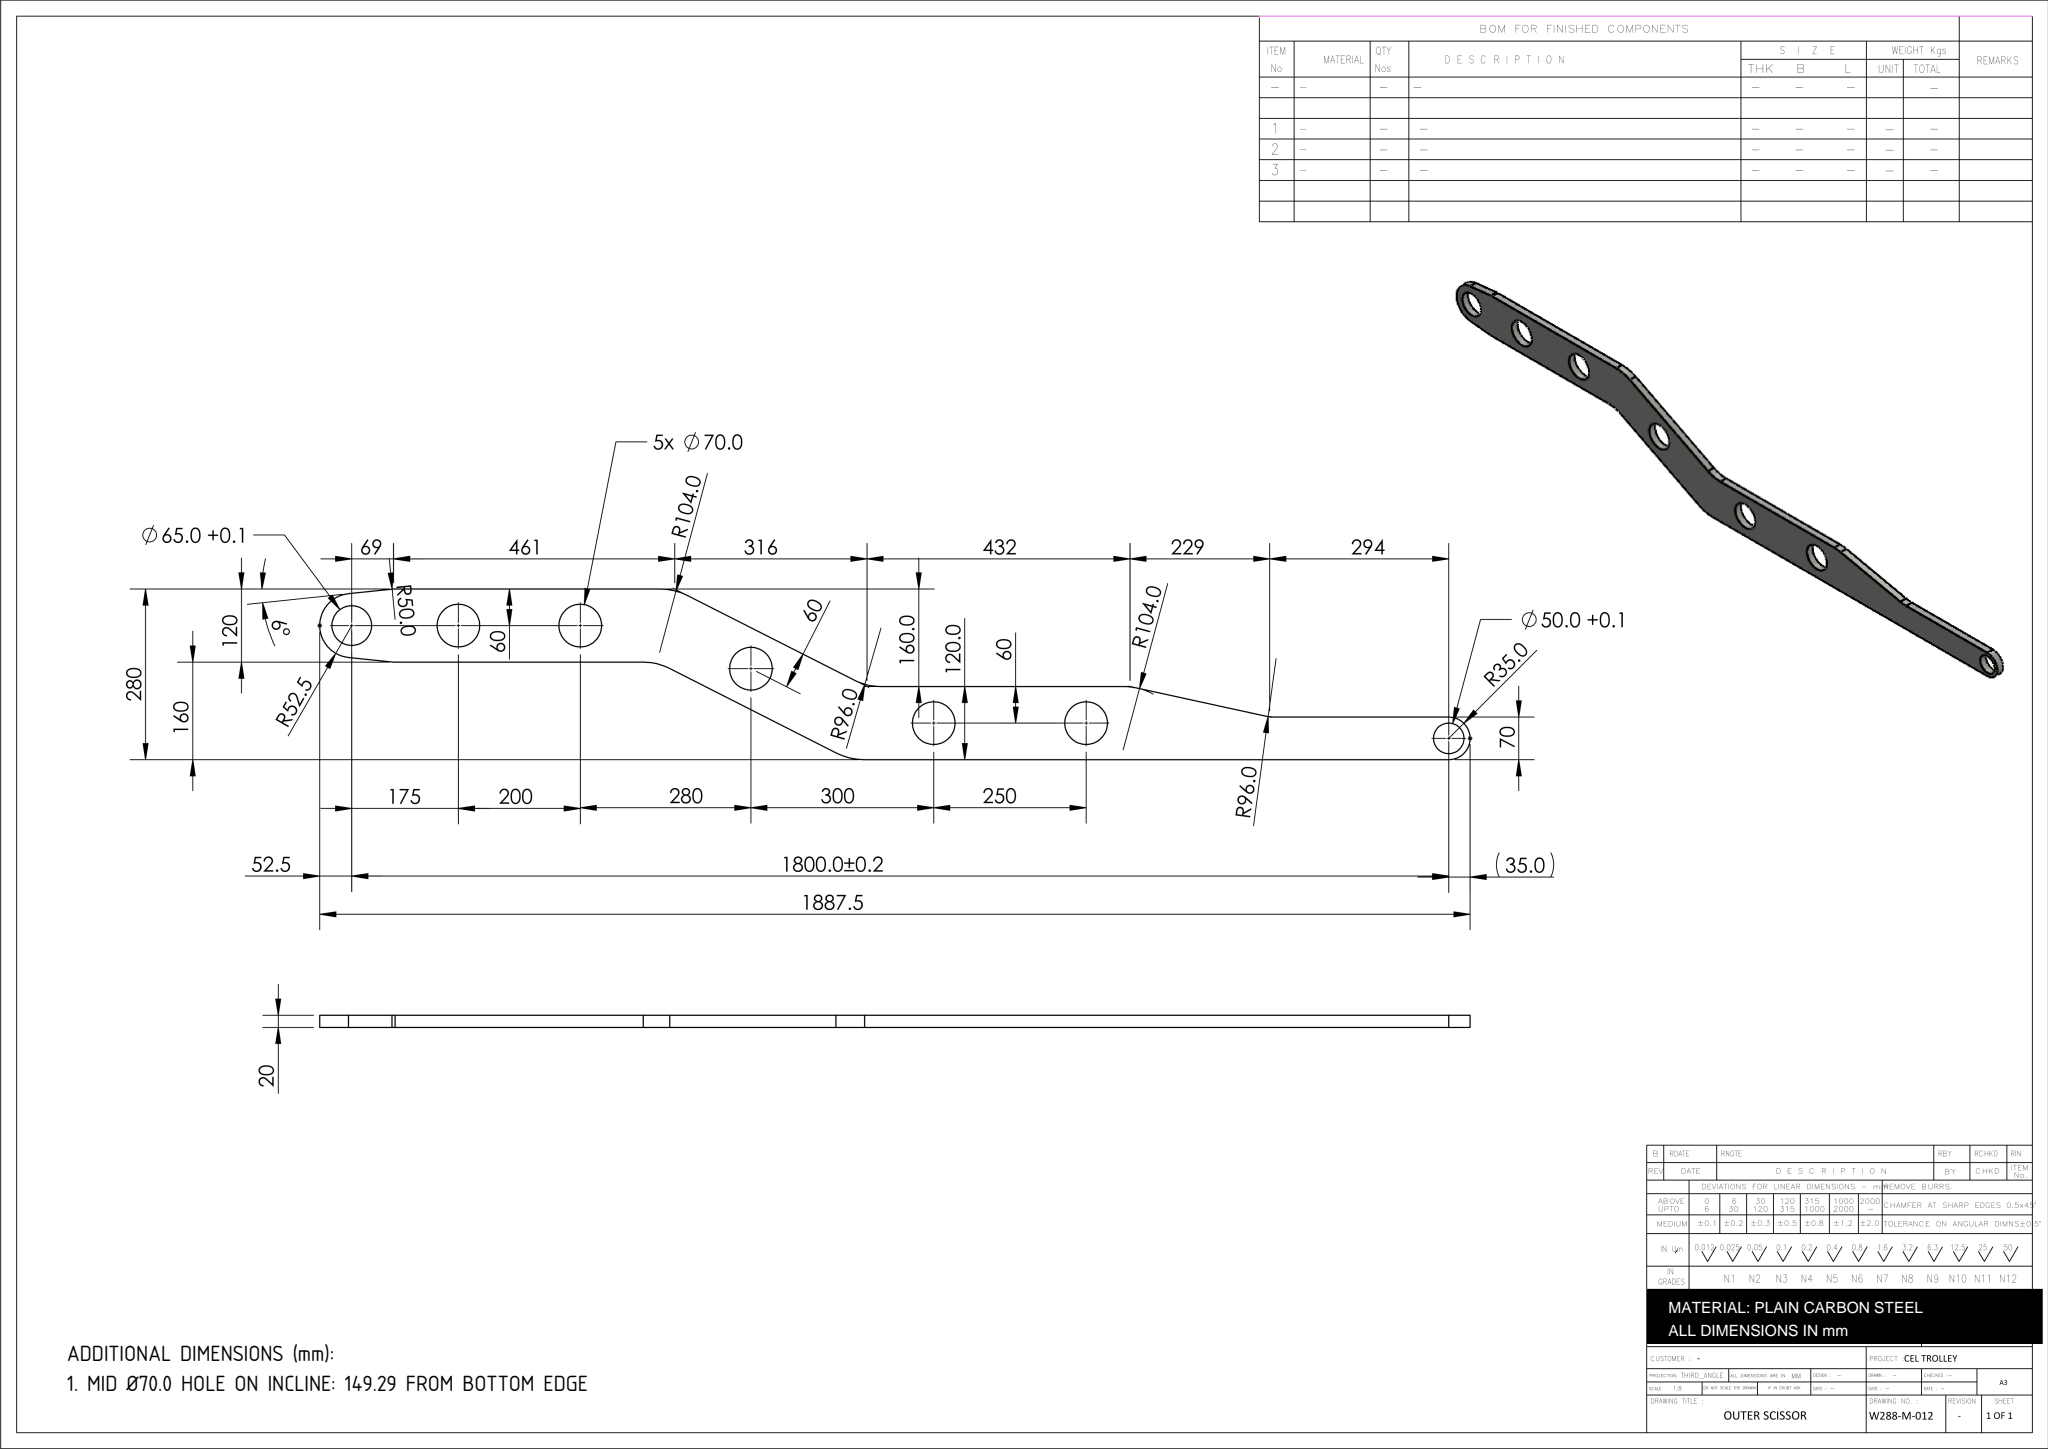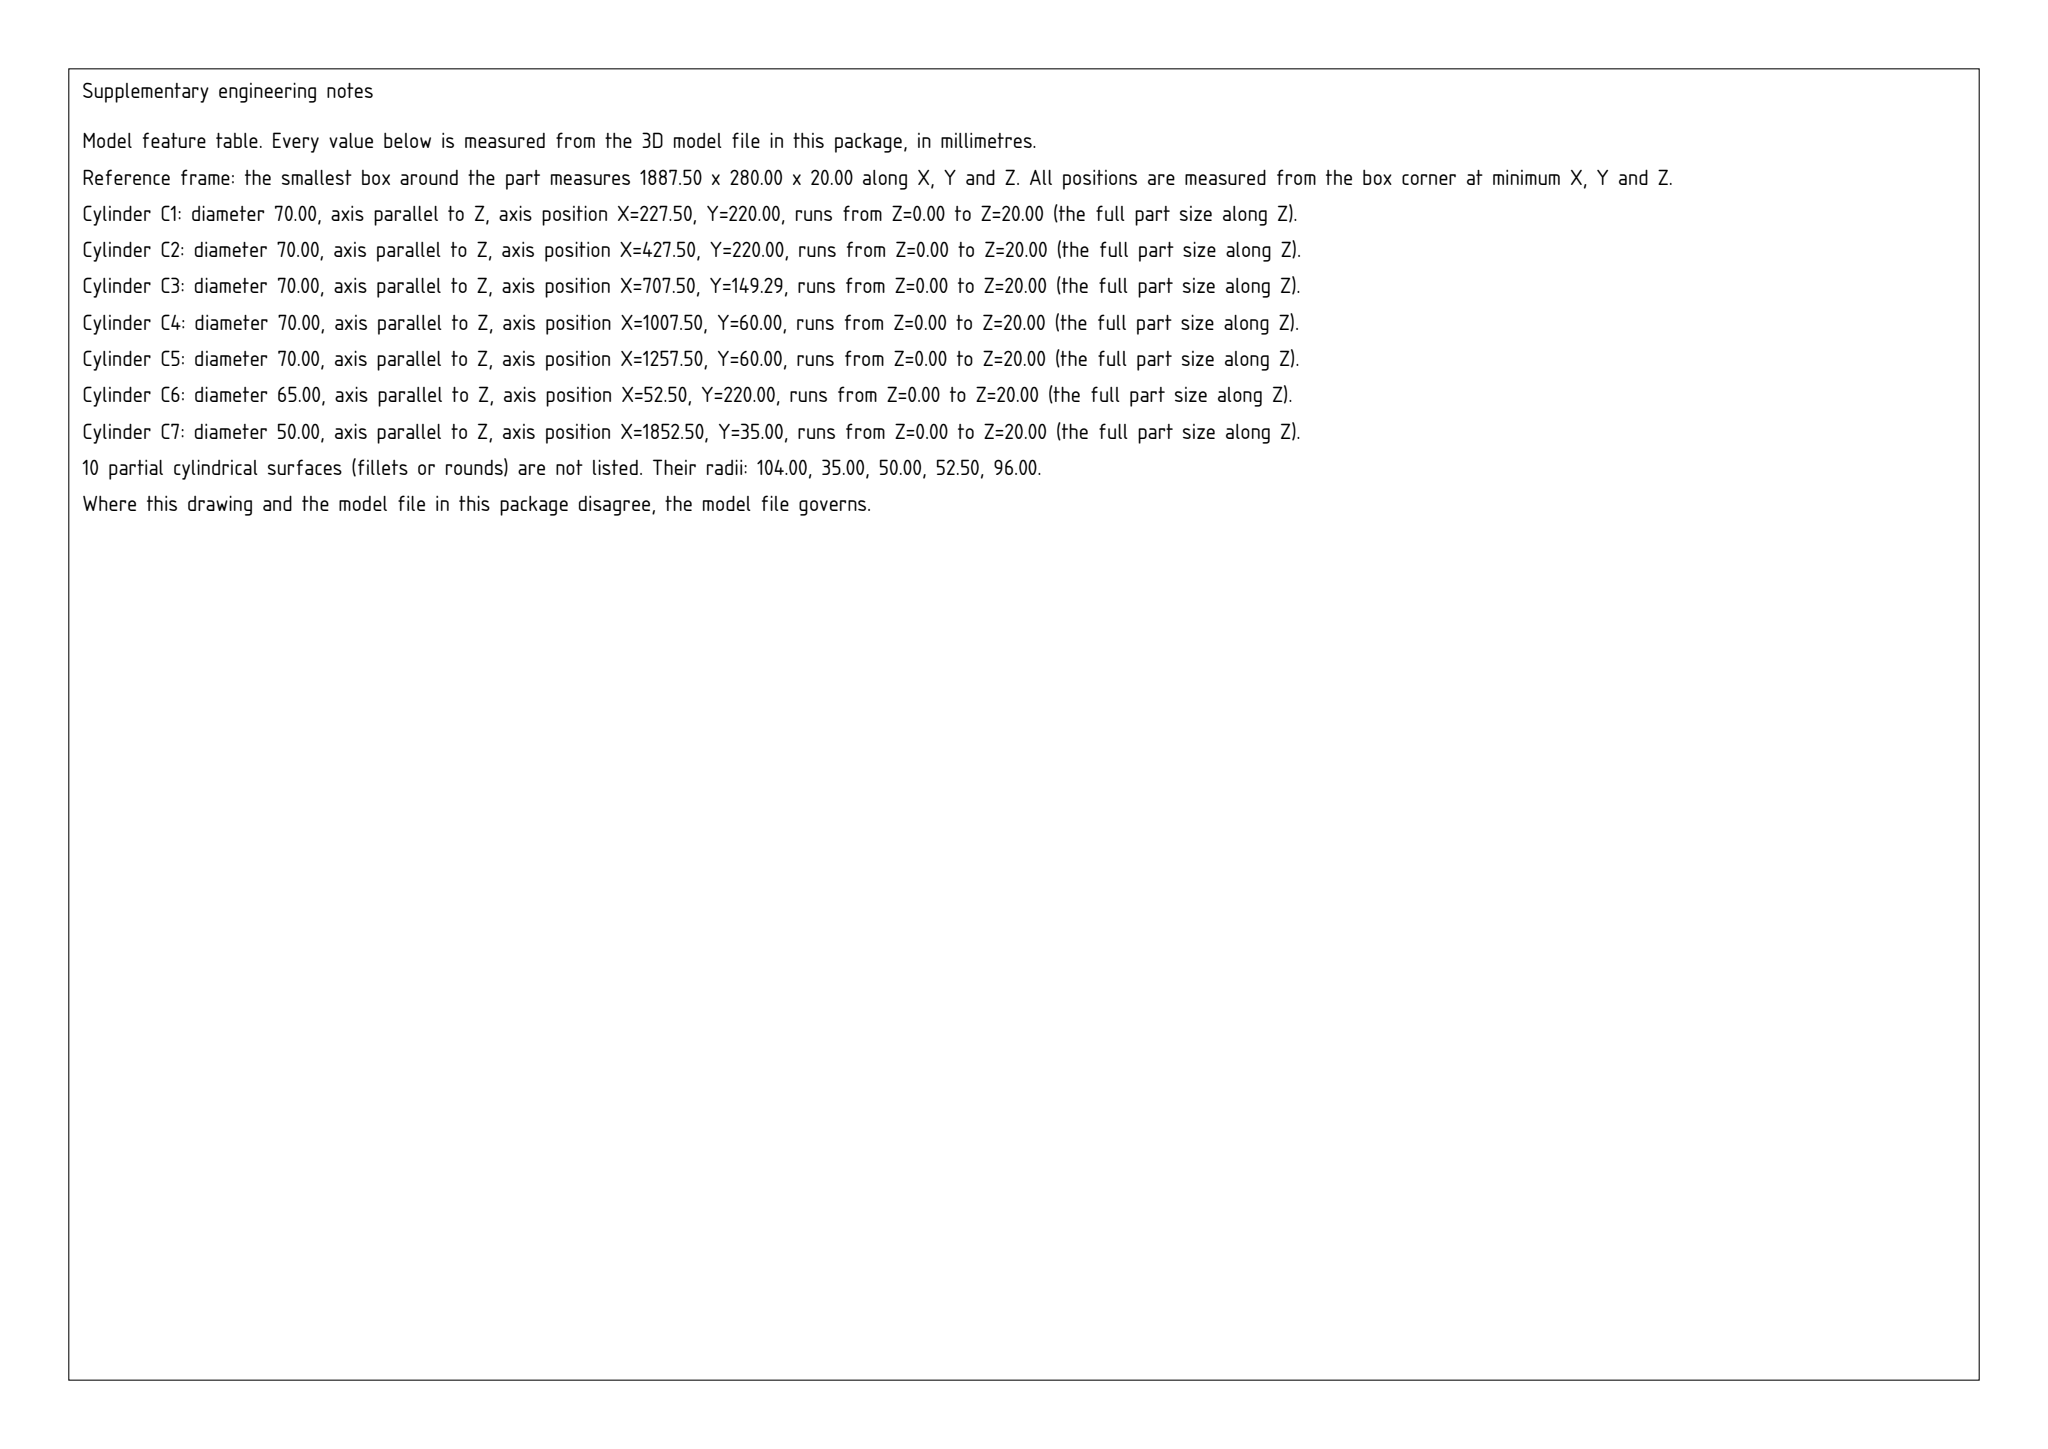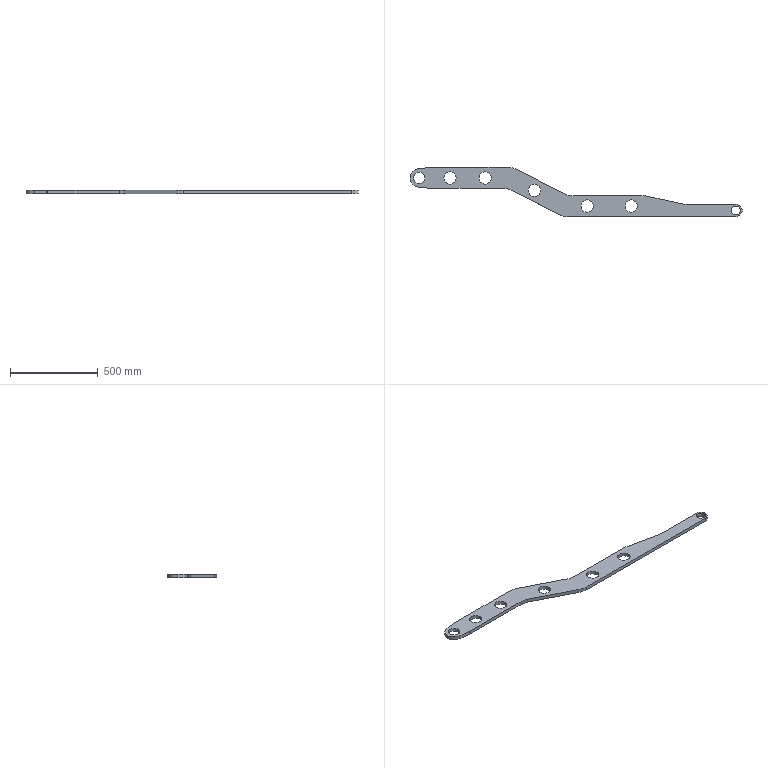Part | SolidWorks | mm | 1 solid | 37 faces | box 1887.5 x 280 x 20 mm | volume 3627831 mm3 | cylinder 25 | plane 12 | commonest cylinder face diameters 70 x11 208 x3 192 x3 50 x2 65 x2 105 x2 100 x2
build123d program:
from build123d import *

# Parameters (mm, degrees)
SKETCH1_R           = 32.5
SKETCH1_R_2         = 25
BOSS_EXTRUDE1_DEPTH = 20
SKETCH3_R           = 35
CUT_EXTRUDE1_DEPTH  = 64


with BuildPart() as part:
    # Sketch1 → Boss-Extrude1 (new body)
    with BuildSketch(Plane.XY):
        with BuildLine():
            Line((119.118, -2.388), (327.362, -47.796))
            ThreePointArc((327.362, -47.796), (337.53, -49.447), (347.815, -50))
            Line((347.815, -50), (631.208, -50))
            ThreePointArc((631.208, -50), (666.208, -85), (631.208, -120))
            Line((631.208, -120), (-327.193, -120))
            ThreePointArc((-327.193, -120), (-351.374, -117.15), (-374.229, -108.756))
            Line((-374.229, -108.756), (-647.108, 29.621))
            ThreePointArc((-647.108, 29.621), (-668.205, 37.369), (-690.526, 40))
            Line((-690.526, 40), (-1097.566, 40))
            ThreePointArc((-1097.566, 40), (-1100.182, 40.069), (-1102.792, 40.274))
            Line((-1102.792, 40.274), (-1174.28, 47.788))
            ThreePointArc((-1174.28, 47.788), (-1221.292, 100), (-1174.28, 152.212))
            Line((-1174.28, 152.212), (-1102.792, 159.726))
            ThreePointArc((-1102.792, 159.726), (-1100.182, 159.931), (-1097.566, 160))
            Line((-1097.566, 160), (-663.751, 160))
            ThreePointArc((-663.751, 160), (-639.571, 157.15), (-616.715, 148.756))
            Line((-616.715, 148.756), (-343.836, 10.379))
            ThreePointArc((-343.836, 10.379), (-322.739, 2.631), (-300.418, 0))
            Line((-300.418, 0), (96.962, 0))
            ThreePointArc((96.962, 0), (108.104, -0.5986), (119.118, -2.388))
        make_face()
        with Locations((-1168.792, 100)):
            Circle(SKETCH1_R, mode=Mode.SUBTRACT)
        with Locations((631.208, -85)):
            Circle(SKETCH1_R_2, mode=Mode.SUBTRACT)
    extrude(amount=BOSS_EXTRUDE1_DEPTH)

    # Sketch3 → Cut-Extrude1 (cut)
    with BuildSketch(Plane.XY.offset(20)):
        with Locations((-993.792, 100)):
            Circle(SKETCH3_R)
        with Locations((-793.792, 100)):
            Circle(SKETCH3_R)
        with Locations((-513.792, 29.29)):
            Circle(SKETCH3_R)
        with Locations((-213.792, -60)):
            Circle(SKETCH3_R)
        with Locations((36.208, -60)):
            Circle(SKETCH3_R)
    extrude(amount=-CUT_EXTRUDE1_DEPTH, mode=Mode.SUBTRACT)


solid = part.part